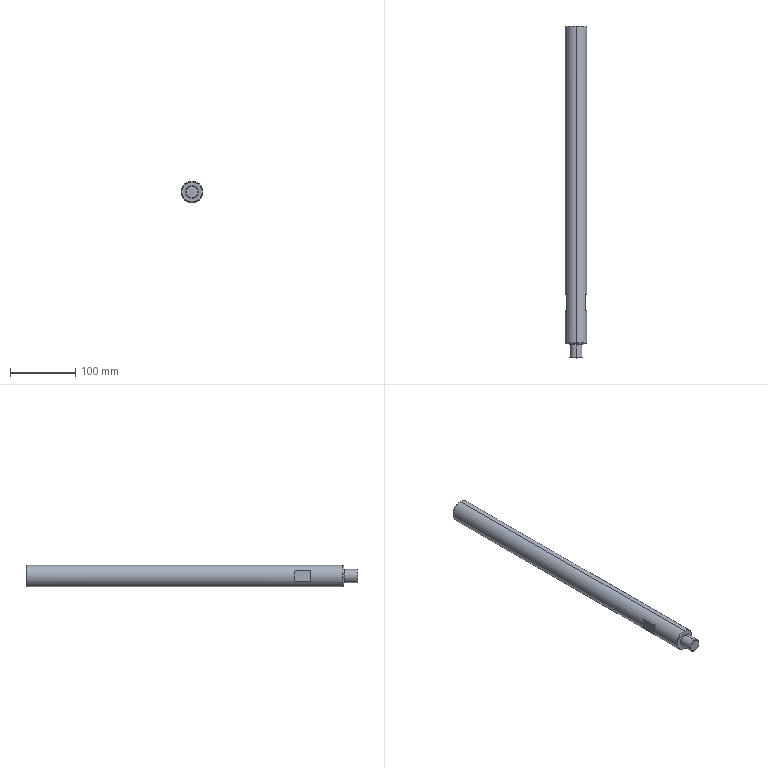Component | SolidWorks | 012A-20130717-1 | 1 solid | 28 faces | box 33 x 508 x 33 mm | volume 408981 mm3 | cone 10 | plane 10 | cylinder 8 | commonest cylinder face diameters 17.5 x2 18 x2 20 x2 33 x2
build123d program:
from build123d import *

# Parameters (mm, degrees)
M20_TAPPED_HOLE1_D     = 17.5
M20_TAPPED_HOLE1_DEPTH = 47.5
M20_TAPPED_HOLE1_TIP   = 5.258
CHAMFER1_SIZE          = 1
CHAMFER2_SIZE          = 1
SKETCH5_OUTSIDE_W      = 137.028
SKETCH5_OUTSIDE_H      = 137.028
SKETCH5_OUTSIDE_W_2    = 41.855
SKETCH5_OUTSIDE_H_2    = 28
CUT_EXTRUDE1_DEPTH     = 25


with BuildPart() as part:
    # Sketch1 → Revolve1 (revolve)
    with BuildSketch(Plane.XY, mode=Mode.PRIVATE) as revolve1_sk:
        Polygon((0, 0), (0, 10), (20, 10), (20, 9), (22, 9), (22, 16.5), (508, 16.5), (508, 0), align=None)
    revolve(revolve1_sk.sketch.rotate(Axis((0, 0, 0), (1, 0, 0)), 90), axis=Axis((0, 0, 0), (1, 0, 0)))

    # M20 Tapped Hole1
    with Locations(Plane(origin=(508, 0, 0), x_dir=(0, 0, 1), z_dir=(1, 0, 0))):
        with Locations((0, 0)):
            Hole(M20_TAPPED_HOLE1_D / 2, depth=M20_TAPPED_HOLE1_DEPTH)
            with Locations((0, 0, -(M20_TAPPED_HOLE1_DEPTH + M20_TAPPED_HOLE1_TIP / 2))):  # 118° drill point
                Cone(0, M20_TAPPED_HOLE1_D / 2, M20_TAPPED_HOLE1_TIP, mode=Mode.SUBTRACT)

    # Chamfer1
    chamfer1_edges = [part.edges().sort_by_distance(p)[0] for p in [
        (0, 0, -10),
    ]]
    chamfer(chamfer1_edges, length=CHAMFER1_SIZE)

    # Chamfer2
    chamfer2_edges = [part.edges().sort_by_distance(p)[0] for p in [
        (508, 0, 8.75),
        (508, 0, -16.5),
        (22, 0, -16.5),
    ]]
    chamfer(chamfer2_edges, length=CHAMFER2_SIZE)

    # Sketch5 outside → Cut-Extrude1 (cut)
    with BuildSketch(Plane.ZY.offset(-72)):
        Rectangle(SKETCH5_OUTSIDE_W, SKETCH5_OUTSIDE_H)
        Rectangle(SKETCH5_OUTSIDE_W_2, SKETCH5_OUTSIDE_H_2, mode=Mode.SUBTRACT)
    extrude(amount=-CUT_EXTRUDE1_DEPTH, mode=Mode.SUBTRACT)


solid = part.part

# Placed as in the assembly
solid = solid.moved(Location((-240, 407.253, 90), (0, 0, 90)))
STEP:
#1=CARTESIAN_POINT('',(-9.449,16.9,4.154));
#2=VERTEX_POINT('',#1);
#3=CARTESIAN_POINT('',(-9.449,16.9,2.933));
#4=VERTEX_POINT('',#3);
#5=CARTESIAN_POINT('',(-9.449,16.9,3.543));
#6=DIRECTION('',(0.,-1.,-0.));
#7=DIRECTION('',(0.,0.,-1.));
#8=AXIS2_PLACEMENT_3D('',#5,#6,#7);
#9=CIRCLE('',#8,0.6102);
#10=EDGE_CURVE('',#2,#4,#9,.T.);
#11=ORIENTED_EDGE('',*,*,#10,.F.);
#12=CARTESIAN_POINT('',(-9.449,16.939,4.193));
#13=VERTEX_POINT('',#12);
#14=CARTESIAN_POINT('',(-9.449,16.9,4.154));
#15=DIRECTION('',(-0.,0.7071,0.7071));
#16=VECTOR('',#15,39.37);
#17=LINE('',#14,#16);
#18=EDGE_CURVE('',#2,#13,#17,.T.);
#19=ORIENTED_EDGE('',*,*,#18,.T.);
#20=CARTESIAN_POINT('',(-9.449,16.939,2.894));
#21=VERTEX_POINT('',#20);
#22=CARTESIAN_POINT('',(-9.449,16.939,3.543));
#23=DIRECTION('',(0.,1.,0.));
#24=DIRECTION('',(0.,0.,-1.));
#25=AXIS2_PLACEMENT_3D('',#22,#23,#24);
#26=CIRCLE('',#25,0.6496);
#27=EDGE_CURVE('',#21,#13,#26,.T.);
#28=ORIENTED_EDGE('',*,*,#27,.F.);
#29=CARTESIAN_POINT('',(-9.449,16.9,2.933));
#30=DIRECTION('',(0.,0.7071,-0.7071));
#31=VECTOR('',#30,39.37);
#32=LINE('',#29,#31);
#33=EDGE_CURVE('',#4,#21,#32,.T.);
#34=ORIENTED_EDGE('',*,*,#33,.F.);
#35=EDGE_LOOP('',(#11,#19,#28,#34));
#36=FACE_OUTER_BOUND('',#35,.T.);
#37=CARTESIAN_POINT('',(-9.449,16.9,3.543));
#38=DIRECTION('',(0.,1.,0.));
#39=DIRECTION('',(0.,0.,-1.));
#40=AXIS2_PLACEMENT_3D('',#37,#38,#39);
#41=CONICAL_SURFACE('',#40,0.6102,0.7854);
#42=ADVANCED_FACE('',(#36),#41,.T.);
#43=CARTESIAN_POINT('',(-9.449,36.034,2.933));
#44=VERTEX_POINT('',#43);
#45=CARTESIAN_POINT('',(-9.449,36.034,4.154));
#46=VERTEX_POINT('',#45);
#47=CARTESIAN_POINT('',(-9.449,36.034,3.543));
#48=DIRECTION('',(0.,1.,0.));
#49=DIRECTION('',(0.,0.,1.));
#50=AXIS2_PLACEMENT_3D('',#47,#48,#49);
#51=CIRCLE('',#50,0.6102);
#52=EDGE_CURVE('',#44,#46,#51,.T.);
#53=ORIENTED_EDGE('',*,*,#52,.F.);
#54=CARTESIAN_POINT('',(-9.449,35.994,2.894));
#55=VERTEX_POINT('',#54);
#56=CARTESIAN_POINT('',(-9.449,35.994,2.894));
#57=DIRECTION('',(-0.,-0.7071,-0.7071));
#58=VECTOR('',#57,39.37);
#59=LINE('',#56,#58);
#60=EDGE_CURVE('',#44,#55,#59,.T.);
#61=ORIENTED_EDGE('',*,*,#60,.T.);
#62=CARTESIAN_POINT('',(-9.449,35.994,4.193));
#63=VERTEX_POINT('',#62);
#64=CARTESIAN_POINT('',(-9.449,35.994,3.543));
#65=DIRECTION('',(0.,-1.,-0.));
#66=DIRECTION('',(0.,0.,1.));
#67=AXIS2_PLACEMENT_3D('',#64,#65,#66);
#68=CIRCLE('',#67,0.6496);
#69=EDGE_CURVE('',#63,#55,#68,.T.);
#70=ORIENTED_EDGE('',*,*,#69,.F.);
#71=CARTESIAN_POINT('',(-9.449,35.994,4.193));
#72=DIRECTION('',(-0.,-0.7071,0.7071));
#73=VECTOR('',#72,39.37);
#74=LINE('',#71,#73);
#75=EDGE_CURVE('',#46,#63,#74,.T.);
#76=ORIENTED_EDGE('',*,*,#75,.F.);
#77=EDGE_LOOP('',(#53,#61,#70,#76));
#78=FACE_OUTER_BOUND('',#77,.T.);
#79=CARTESIAN_POINT('',(-9.449,35.994,3.543));
#80=DIRECTION('',(0.,-1.,-0.));
#81=DIRECTION('',(0.,0.,1.));
#82=AXIS2_PLACEMENT_3D('',#79,#80,#81);
#83=CONICAL_SURFACE('',#82,0.6496,0.7854);
#84=ADVANCED_FACE('',(#78),#83,.T.);
#85=CARTESIAN_POINT('',(-9.449,35.994,3.888));
#86=VERTEX_POINT('',#85);
#87=CARTESIAN_POINT('',(-9.449,35.994,3.199));
#88=VERTEX_POINT('',#87);
#89=CARTESIAN_POINT('',(-9.449,35.994,3.543));
#90=DIRECTION('',(0.,1.,0.));
#91=DIRECTION('',(0.,0.,1.));
#92=AXIS2_PLACEMENT_3D('',#89,#90,#91);
#93=CIRCLE('',#92,0.3445);
#94=EDGE_CURVE('',#86,#88,#93,.T.);
#95=ORIENTED_EDGE('',*,*,#94,.F.);
#96=CARTESIAN_POINT('',(-9.449,36.034,3.927));
#97=VERTEX_POINT('',#96);
#98=CARTESIAN_POINT('',(-9.449,35.994,3.888));
#99=DIRECTION('',(-0.,0.7071,0.7071));
#100=VECTOR('',#99,39.37);
#101=LINE('',#98,#100);
#102=EDGE_CURVE('',#86,#97,#101,.T.);
#103=ORIENTED_EDGE('',*,*,#102,.T.);
#104=CARTESIAN_POINT('',(-9.449,36.034,3.159));
#105=VERTEX_POINT('',#104);
#106=CARTESIAN_POINT('',(-9.449,36.034,3.543));
#107=DIRECTION('',(0.,-1.,-0.));
#108=DIRECTION('',(0.,0.,1.));
#109=AXIS2_PLACEMENT_3D('',#106,#107,#108);
#110=CIRCLE('',#109,0.3839);
#111=EDGE_CURVE('',#105,#97,#110,.T.);
#112=ORIENTED_EDGE('',*,*,#111,.F.);
#113=CARTESIAN_POINT('',(-9.449,35.994,3.199));
#114=DIRECTION('',(0.,0.7071,-0.7071));
#115=VECTOR('',#114,39.37);
#116=LINE('',#113,#115);
#117=EDGE_CURVE('',#88,#105,#116,.T.);
#118=ORIENTED_EDGE('',*,*,#117,.F.);
#119=EDGE_LOOP('',(#95,#103,#112,#118));
#120=FACE_OUTER_BOUND('',#119,.T.);
#121=CARTESIAN_POINT('',(-9.449,35.994,3.543));
#122=DIRECTION('',(0.,1.,0.));
#123=DIRECTION('',(0.,0.,-1.));
#124=AXIS2_PLACEMENT_3D('',#121,#122,#123);
#125=CONICAL_SURFACE('',#124,0.3445,0.7854);
#126=ADVANCED_FACE('',(#120),#125,.F.);
#127=CARTESIAN_POINT('',(-9.449,16.034,3.898));
#128=VERTEX_POINT('',#127);
#129=CARTESIAN_POINT('',(-9.449,16.034,3.189));
#130=VERTEX_POINT('',#129);
#131=CARTESIAN_POINT('',(-9.449,16.034,3.543));
#132=DIRECTION('',(0.,-1.,-0.));
#133=DIRECTION('',(0.,0.,-1.));
#134=AXIS2_PLACEMENT_3D('',#131,#132,#133);
#135=CIRCLE('',#134,0.3543);
#136=EDGE_CURVE('',#128,#130,#135,.T.);
#137=ORIENTED_EDGE('',*,*,#136,.F.);
#138=CARTESIAN_POINT('',(-9.449,16.073,3.937));
#139=VERTEX_POINT('',#138);
#140=CARTESIAN_POINT('',(-9.449,16.034,3.898));
#141=DIRECTION('',(-0.,0.7071,0.7071));
#142=VECTOR('',#141,39.37);
#143=LINE('',#140,#142);
#144=EDGE_CURVE('',#128,#139,#143,.T.);
#145=ORIENTED_EDGE('',*,*,#144,.T.);
#146=CARTESIAN_POINT('',(-9.449,16.073,3.15));
#147=VERTEX_POINT('',#146);
#148=CARTESIAN_POINT('',(-9.449,16.073,3.543));
#149=DIRECTION('',(0.,1.,0.));
#150=DIRECTION('',(0.,0.,-1.));
#151=AXIS2_PLACEMENT_3D('',#148,#149,#150);
#152=CIRCLE('',#151,0.3937);
#153=EDGE_CURVE('',#147,#139,#152,.T.);
#154=ORIENTED_EDGE('',*,*,#153,.F.);
#155=CARTESIAN_POINT('',(-9.449,16.034,3.189));
#156=DIRECTION('',(0.,0.7071,-0.7071));
#157=VECTOR('',#156,39.37);
#158=LINE('',#155,#157);
#159=EDGE_CURVE('',#130,#147,#158,.T.);
#160=ORIENTED_EDGE('',*,*,#159,.F.);
#161=EDGE_LOOP('',(#137,#145,#154,#160));
#162=FACE_OUTER_BOUND('',#161,.T.);
#163=CARTESIAN_POINT('',(-9.449,16.034,3.543));
#164=DIRECTION('',(0.,1.,0.));
#165=DIRECTION('',(0.,0.,-1.));
#166=AXIS2_PLACEMENT_3D('',#163,#164,#165);
#167=CONICAL_SURFACE('',#166,0.3543,0.7854);
#168=ADVANCED_FACE('',(#162),#167,.T.);
#169=CARTESIAN_POINT('',(-9.449,34.164,3.888));
#170=VERTEX_POINT('',#169);
#171=CARTESIAN_POINT('',(-9.449,34.164,3.199));
#172=VERTEX_POINT('',#171);
#173=CARTESIAN_POINT('',(-9.449,34.164,3.543));
#174=DIRECTION('',(0.,1.,0.));
#175=DIRECTION('',(0.,0.,-1.));
#176=AXIS2_PLACEMENT_3D('',#173,#174,#175);
#177=CIRCLE('',#176,0.3445);
#178=EDGE_CURVE('',#170,#172,#177,.T.);
#179=ORIENTED_EDGE('',*,*,#178,.F.);
#180=CARTESIAN_POINT('',(-9.449,36.034,3.888));
#181=DIRECTION('',(0.,1.,0.));
#182=VECTOR('',#181,39.37);
#183=LINE('',#180,#182);
#184=EDGE_CURVE('',#170,#86,#183,.T.);
#185=ORIENTED_EDGE('',*,*,#184,.T.);
#186=ORIENTED_EDGE('',*,*,#94,.T.);
#187=CARTESIAN_POINT('',(-9.449,36.034,3.199));
#188=DIRECTION('',(0.,1.,0.));
#189=VECTOR('',#188,39.37);
#190=LINE('',#187,#189);
#191=EDGE_CURVE('',#172,#88,#190,.T.);
#192=ORIENTED_EDGE('',*,*,#191,.F.);
#193=EDGE_LOOP('',(#179,#185,#186,#192));
#194=FACE_OUTER_BOUND('',#193,.T.);
#195=CARTESIAN_POINT('',(-9.449,36.034,3.543));
#196=DIRECTION('',(0.,1.,0.));
#197=DIRECTION('',(0.,0.,-1.));
#198=AXIS2_PLACEMENT_3D('',#195,#196,#197);
#199=CYLINDRICAL_SURFACE('',#198,0.3445);
#200=ADVANCED_FACE('',(#194),#199,.F.);
#201=CARTESIAN_POINT('',(-9.449,33.957,3.543));
#202=VERTEX_POINT('',#201);
#203=CARTESIAN_POINT('',(-9.449,34.164,3.199));
#204=DIRECTION('',(0.,0.515,-0.8572));
#205=VECTOR('',#204,39.37);
#206=LINE('',#203,#205);
#207=EDGE_CURVE('',#202,#172,#206,.T.);
#208=ORIENTED_EDGE('',*,*,#207,.F.);
#209=CARTESIAN_POINT('',(-9.449,34.164,3.888));
#210=DIRECTION('',(-0.,0.515,0.8572));
#211=VECTOR('',#210,39.37);
#212=LINE('',#209,#211);
#213=EDGE_CURVE('',#202,#170,#212,.T.);
#214=ORIENTED_EDGE('',*,*,#213,.T.);
#215=ORIENTED_EDGE('',*,*,#178,.T.);
#216=EDGE_LOOP('',(#208,#214,#215));
#217=FACE_OUTER_BOUND('',#216,.T.);
#218=CARTESIAN_POINT('',(-9.449,34.164,3.543));
#219=DIRECTION('',(0.,1.,0.));
#220=DIRECTION('',(0.,0.,-1.));
#221=AXIS2_PLACEMENT_3D('',#218,#219,#220);
#222=CONICAL_SURFACE('',#221,0.3445,1.03);
#223=ADVANCED_FACE('',(#217),#222,.F.);
#224=CARTESIAN_POINT('',(-9.449,16.9,3.898));
#225=VERTEX_POINT('',#224);
#226=CARTESIAN_POINT('',(-9.449,16.9,3.189));
#227=VERTEX_POINT('',#226);
#228=CARTESIAN_POINT('',(-9.449,16.9,3.543));
#229=DIRECTION('',(0.,-1.,-0.));
#230=DIRECTION('',(0.,0.,1.));
#231=AXIS2_PLACEMENT_3D('',#228,#229,#230);
#232=CIRCLE('',#231,0.3543);
#233=EDGE_CURVE('',#225,#227,#232,.T.);
#234=ORIENTED_EDGE('',*,*,#233,.T.);
#235=CARTESIAN_POINT('',(-9.449,16.821,3.189));
#236=VERTEX_POINT('',#235);
#237=CARTESIAN_POINT('',(-9.449,16.034,3.189));
#238=DIRECTION('',(0.,-1.,-0.));
#239=VECTOR('',#238,39.37);
#240=LINE('',#237,#239);
#241=EDGE_CURVE('',#227,#236,#240,.T.);
#242=ORIENTED_EDGE('',*,*,#241,.T.);
#243=CARTESIAN_POINT('',(-9.449,16.821,3.898));
#244=VERTEX_POINT('',#243);
#245=CARTESIAN_POINT('',(-9.449,16.821,3.543));
#246=DIRECTION('',(0.,-1.,-0.));
#247=DIRECTION('',(0.,0.,1.));
#248=AXIS2_PLACEMENT_3D('',#245,#246,#247);
#249=CIRCLE('',#248,0.3543);
#250=EDGE_CURVE('',#244,#236,#249,.T.);
#251=ORIENTED_EDGE('',*,*,#250,.F.);
#252=CARTESIAN_POINT('',(-9.449,16.034,3.898));
#253=DIRECTION('',(0.,-1.,-0.));
#254=VECTOR('',#253,39.37);
#255=LINE('',#252,#254);
#256=EDGE_CURVE('',#225,#244,#255,.T.);
#257=ORIENTED_EDGE('',*,*,#256,.F.);
#258=EDGE_LOOP('',(#234,#242,#251,#257));
#259=FACE_OUTER_BOUND('',#258,.T.);
#260=CARTESIAN_POINT('',(-9.449,16.034,3.543));
#261=DIRECTION('',(0.,-1.,-0.));
#262=DIRECTION('',(0.,0.,1.));
#263=AXIS2_PLACEMENT_3D('',#260,#261,#262);
#264=CYLINDRICAL_SURFACE('',#263,0.3543);
#265=ADVANCED_FACE('',(#259),#264,.T.);
#266=CARTESIAN_POINT('',(-9.449,16.821,3.937));
#267=VERTEX_POINT('',#266);
#268=CARTESIAN_POINT('',(-9.449,16.821,3.15));
#269=VERTEX_POINT('',#268);
#270=CARTESIAN_POINT('',(-9.449,16.821,3.543));
#271=DIRECTION('',(0.,-1.,-0.));
#272=DIRECTION('',(0.,0.,1.));
#273=AXIS2_PLACEMENT_3D('',#270,#271,#272);
#274=CIRCLE('',#273,0.3937);
#275=EDGE_CURVE('',#267,#269,#274,.T.);
#276=ORIENTED_EDGE('',*,*,#275,.T.);
#277=CARTESIAN_POINT('',(-9.449,16.034,3.15));
#278=DIRECTION('',(0.,-1.,-0.));
#279=VECTOR('',#278,39.37);
#280=LINE('',#277,#279);
#281=EDGE_CURVE('',#269,#147,#280,.T.);
#282=ORIENTED_EDGE('',*,*,#281,.T.);
#283=ORIENTED_EDGE('',*,*,#153,.T.);
#284=CARTESIAN_POINT('',(-9.449,16.034,3.937));
#285=DIRECTION('',(0.,-1.,-0.));
#286=VECTOR('',#285,39.37);
#287=LINE('',#284,#286);
#288=EDGE_CURVE('',#267,#139,#287,.T.);
#289=ORIENTED_EDGE('',*,*,#288,.F.);
#290=EDGE_LOOP('',(#276,#282,#283,#289));
#291=FACE_OUTER_BOUND('',#290,.T.);
#292=CARTESIAN_POINT('',(-9.449,16.034,3.543));
#293=DIRECTION('',(0.,-1.,-0.));
#294=DIRECTION('',(0.,0.,1.));
#295=AXIS2_PLACEMENT_3D('',#292,#293,#294);
#296=CYLINDRICAL_SURFACE('',#295,0.3937);
#297=ADVANCED_FACE('',(#291),#296,.T.);
#298=CARTESIAN_POINT('',(-10.,19.852,3.2));
#299=VERTEX_POINT('',#298);
#300=CARTESIAN_POINT('',(-10.,18.868,3.2));
#301=VERTEX_POINT('',#300);
#302=CARTESIAN_POINT('',(-10.,16.034,3.2));
#303=DIRECTION('',(0.,-1.,-0.));
#304=VECTOR('',#303,39.37);
#305=LINE('',#302,#304);
#306=EDGE_CURVE('',#299,#301,#305,.T.);
#307=ORIENTED_EDGE('',*,*,#306,.F.);
#308=CARTESIAN_POINT('',(-10.,19.852,3.887));
#309=VERTEX_POINT('',#308);
#310=CARTESIAN_POINT('',(-9.449,19.852,3.543));
#311=DIRECTION('',(0.,-1.,-0.));
#312=DIRECTION('',(0.,0.,1.));
#313=AXIS2_PLACEMENT_3D('',#310,#311,#312);
#314=CIRCLE('',#313,0.6496);
#315=EDGE_CURVE('',#309,#299,#314,.T.);
#316=ORIENTED_EDGE('',*,*,#315,.F.);
#317=CARTESIAN_POINT('',(-10.,18.868,3.887));
#318=VERTEX_POINT('',#317);
#319=CARTESIAN_POINT('',(-10.,16.034,3.887));
#320=DIRECTION('',(0.,1.,0.));
#321=VECTOR('',#320,39.37);
#322=LINE('',#319,#321);
#323=EDGE_CURVE('',#318,#309,#322,.T.);
#324=ORIENTED_EDGE('',*,*,#323,.F.);
#325=CARTESIAN_POINT('',(-9.449,18.868,3.543));
#326=DIRECTION('',(0.,-1.,-0.));
#327=DIRECTION('',(0.,0.,1.));
#328=AXIS2_PLACEMENT_3D('',#325,#326,#327);
#329=CIRCLE('',#328,0.6496);
#330=EDGE_CURVE('',#318,#301,#329,.T.);
#331=ORIENTED_EDGE('',*,*,#330,.T.);
#332=EDGE_LOOP('',(#307,#316,#324,#331));
#333=FACE_BOUND('',#332,.T.);
#334=ORIENTED_EDGE('',*,*,#69,.T.);
#335=CARTESIAN_POINT('',(-9.449,16.034,2.894));
#336=DIRECTION('',(0.,-1.,-0.));
#337=VECTOR('',#336,39.37);
#338=LINE('',#335,#337);
#339=EDGE_CURVE('',#55,#21,#338,.T.);
#340=ORIENTED_EDGE('',*,*,#339,.T.);
#341=ORIENTED_EDGE('',*,*,#27,.T.);
#342=CARTESIAN_POINT('',(-9.449,16.034,4.193));
#343=DIRECTION('',(0.,-1.,-0.));
#344=VECTOR('',#343,39.37);
#345=LINE('',#342,#344);
#346=EDGE_CURVE('',#63,#13,#345,.T.);
#347=ORIENTED_EDGE('',*,*,#346,.F.);
#348=EDGE_LOOP('',(#334,#340,#341,#347));
#349=FACE_OUTER_BOUND('',#348,.T.);
#350=CARTESIAN_POINT('',(-9.449,16.034,3.543));
#351=DIRECTION('',(0.,-1.,-0.));
#352=DIRECTION('',(0.,0.,1.));
#353=AXIS2_PLACEMENT_3D('',#350,#351,#352);
#354=CYLINDRICAL_SURFACE('',#353,0.6496);
#355=ADVANCED_FACE('',(#333,#349),#354,.T.);
#356=ORIENTED_EDGE('',*,*,#339,.F.);
#357=CARTESIAN_POINT('',(-9.449,35.994,3.543));
#358=DIRECTION('',(0.,-1.,-0.));
#359=DIRECTION('',(0.,0.,1.));
#360=AXIS2_PLACEMENT_3D('',#357,#358,#359);
#361=CIRCLE('',#360,0.6496);
#362=EDGE_CURVE('',#55,#63,#361,.T.);
#363=ORIENTED_EDGE('',*,*,#362,.T.);
#364=ORIENTED_EDGE('',*,*,#346,.T.);
#365=CARTESIAN_POINT('',(-9.449,16.939,3.543));
#366=DIRECTION('',(0.,1.,0.));
#367=DIRECTION('',(0.,0.,-1.));
#368=AXIS2_PLACEMENT_3D('',#365,#366,#367);
#369=CIRCLE('',#368,0.6496);
#370=EDGE_CURVE('',#13,#21,#369,.T.);
#371=ORIENTED_EDGE('',*,*,#370,.T.);
#372=EDGE_LOOP('',(#356,#363,#364,#371));
#373=FACE_OUTER_BOUND('',#372,.T.);
#374=CARTESIAN_POINT('',(-8.898,19.852,3.887));
#375=VERTEX_POINT('',#374);
#376=CARTESIAN_POINT('',(-8.898,18.868,3.887));
#377=VERTEX_POINT('',#376);
#378=CARTESIAN_POINT('',(-8.898,16.034,3.887));
#379=DIRECTION('',(0.,-1.,-0.));
#380=VECTOR('',#379,39.37);
#381=LINE('',#378,#380);
#382=EDGE_CURVE('',#375,#377,#381,.T.);
#383=ORIENTED_EDGE('',*,*,#382,.F.);
#384=CARTESIAN_POINT('',(-8.898,19.852,3.2));
#385=VERTEX_POINT('',#384);
#386=CARTESIAN_POINT('',(-9.449,19.852,3.543));
#387=DIRECTION('',(0.,-1.,-0.));
#388=DIRECTION('',(0.,0.,1.));
#389=AXIS2_PLACEMENT_3D('',#386,#387,#388);
#390=CIRCLE('',#389,0.6496);
#391=EDGE_CURVE('',#385,#375,#390,.T.);
#392=ORIENTED_EDGE('',*,*,#391,.F.);
#393=CARTESIAN_POINT('',(-8.898,18.868,3.2));
#394=VERTEX_POINT('',#393);
#395=CARTESIAN_POINT('',(-8.898,16.034,3.2));
#396=DIRECTION('',(0.,1.,0.));
#397=VECTOR('',#396,39.37);
#398=LINE('',#395,#397);
#399=EDGE_CURVE('',#394,#385,#398,.T.);
#400=ORIENTED_EDGE('',*,*,#399,.F.);
#401=CARTESIAN_POINT('',(-9.449,18.868,3.543));
#402=DIRECTION('',(0.,-1.,-0.));
#403=DIRECTION('',(0.,0.,1.));
#404=AXIS2_PLACEMENT_3D('',#401,#402,#403);
#405=CIRCLE('',#404,0.6496);
#406=EDGE_CURVE('',#394,#377,#405,.T.);
#407=ORIENTED_EDGE('',*,*,#406,.T.);
#408=EDGE_LOOP('',(#383,#392,#400,#407));
#409=FACE_BOUND('',#408,.T.);
#410=CARTESIAN_POINT('',(-9.449,16.034,3.543));
#411=DIRECTION('',(0.,-1.,-0.));
#412=DIRECTION('',(0.,0.,1.));
#413=AXIS2_PLACEMENT_3D('',#410,#411,#412);
#414=CYLINDRICAL_SURFACE('',#413,0.6496);
#415=ADVANCED_FACE('',(#373,#409),#414,.T.);
#416=CARTESIAN_POINT('',(-9.449,16.034,3.543));
#417=DIRECTION('',(0.,-1.,-0.));
#418=DIRECTION('',(0.,0.,-1.));
#419=AXIS2_PLACEMENT_3D('',#416,#417,#418);
#420=CIRCLE('',#419,0.3543);
#421=EDGE_CURVE('',#130,#128,#420,.T.);
#422=ORIENTED_EDGE('',*,*,#421,.T.);
#423=ORIENTED_EDGE('',*,*,#136,.T.);
#424=EDGE_LOOP('',(#422,#423));
#425=FACE_OUTER_BOUND('',#424,.T.);
#426=CARTESIAN_POINT('',(-9.449,16.034,3.543));
#427=DIRECTION('',(0.,1.,0.));
#428=DIRECTION('',(0.,0.,-1.));
#429=AXIS2_PLACEMENT_3D('',#426,#427,#428);
#430=PLANE('',#429);
#431=ADVANCED_FACE('',(#425),#430,.F.);
#432=ORIENTED_EDGE('',*,*,#281,.F.);
#433=CARTESIAN_POINT('',(-9.449,16.821,3.543));
#434=DIRECTION('',(0.,-1.,-0.));
#435=DIRECTION('',(0.,0.,1.));
#436=AXIS2_PLACEMENT_3D('',#433,#434,#435);
#437=CIRCLE('',#436,0.3937);
#438=EDGE_CURVE('',#269,#267,#437,.T.);
#439=ORIENTED_EDGE('',*,*,#438,.T.);
#440=ORIENTED_EDGE('',*,*,#288,.T.);
#441=CARTESIAN_POINT('',(-9.449,16.073,3.543));
#442=DIRECTION('',(0.,1.,0.));
#443=DIRECTION('',(0.,0.,-1.));
#444=AXIS2_PLACEMENT_3D('',#441,#442,#443);
#445=CIRCLE('',#444,0.3937);
#446=EDGE_CURVE('',#139,#147,#445,.T.);
#447=ORIENTED_EDGE('',*,*,#446,.T.);
#448=EDGE_LOOP('',(#432,#439,#440,#447));
#449=FACE_OUTER_BOUND('',#448,.T.);
#450=CARTESIAN_POINT('',(-9.449,16.034,3.543));
#451=DIRECTION('',(0.,-1.,-0.));
#452=DIRECTION('',(0.,0.,1.));
#453=AXIS2_PLACEMENT_3D('',#450,#451,#452);
#454=CYLINDRICAL_SURFACE('',#453,0.3937);
#455=ADVANCED_FACE('',(#449),#454,.T.);
#456=ORIENTED_EDGE('',*,*,#275,.F.);
#457=ORIENTED_EDGE('',*,*,#438,.F.);
#458=EDGE_LOOP('',(#456,#457));
#459=FACE_OUTER_BOUND('',#458,.T.);
#460=ORIENTED_EDGE('',*,*,#250,.T.);
#461=CARTESIAN_POINT('',(-9.449,16.821,3.543));
#462=DIRECTION('',(0.,-1.,-0.));
#463=DIRECTION('',(0.,0.,1.));
#464=AXIS2_PLACEMENT_3D('',#461,#462,#463);
#465=CIRCLE('',#464,0.3543);
#466=EDGE_CURVE('',#236,#244,#465,.T.);
#467=ORIENTED_EDGE('',*,*,#466,.T.);
#468=EDGE_LOOP('',(#460,#467));
#469=FACE_BOUND('',#468,.T.);
#470=CARTESIAN_POINT('',(-9.843,16.821,3.543));
#471=DIRECTION('',(0.,-1.,-0.));
#472=DIRECTION('',(-0.,-0.,1.));
#473=AXIS2_PLACEMENT_3D('',#470,#471,#472);
#474=PLANE('',#473);
#475=ADVANCED_FACE('',(#459,#469),#474,.F.);
#476=ORIENTED_EDGE('',*,*,#241,.F.);
#477=CARTESIAN_POINT('',(-9.449,16.9,3.543));
#478=DIRECTION('',(0.,-1.,-0.));
#479=DIRECTION('',(0.,0.,1.));
#480=AXIS2_PLACEMENT_3D('',#477,#478,#479);
#481=CIRCLE('',#480,0.3543);
#482=EDGE_CURVE('',#227,#225,#481,.T.);
#483=ORIENTED_EDGE('',*,*,#482,.T.);
#484=ORIENTED_EDGE('',*,*,#256,.T.);
#485=ORIENTED_EDGE('',*,*,#466,.F.);
#486=EDGE_LOOP('',(#476,#483,#484,#485));
#487=FACE_OUTER_BOUND('',#486,.T.);
#488=CARTESIAN_POINT('',(-9.449,16.034,3.543));
#489=DIRECTION('',(0.,-1.,-0.));
#490=DIRECTION('',(0.,0.,1.));
#491=AXIS2_PLACEMENT_3D('',#488,#489,#490);
#492=CYLINDRICAL_SURFACE('',#491,0.3543);
#493=ADVANCED_FACE('',(#487),#492,.T.);
#494=CARTESIAN_POINT('',(-9.449,16.9,3.543));
#495=DIRECTION('',(0.,-1.,-0.));
#496=DIRECTION('',(0.,0.,-1.));
#497=AXIS2_PLACEMENT_3D('',#494,#495,#496);
#498=CIRCLE('',#497,0.6102);
#499=EDGE_CURVE('',#4,#2,#498,.T.);
#500=ORIENTED_EDGE('',*,*,#499,.T.);
#501=ORIENTED_EDGE('',*,*,#10,.T.);
#502=EDGE_LOOP('',(#500,#501));
#503=FACE_OUTER_BOUND('',#502,.T.);
#504=ORIENTED_EDGE('',*,*,#233,.F.);
#505=ORIENTED_EDGE('',*,*,#482,.F.);
#506=EDGE_LOOP('',(#504,#505));
#507=FACE_BOUND('',#506,.T.);
#508=CARTESIAN_POINT('',(-9.803,16.9,3.543));
#509=DIRECTION('',(0.,1.,0.));
#510=DIRECTION('',(0.,0.,-1.));
#511=AXIS2_PLACEMENT_3D('',#508,#509,#510);
#512=PLANE('',#511);
#513=ADVANCED_FACE('',(#503,#507),#512,.F.);
#514=ORIENTED_EDGE('',*,*,#111,.T.);
#515=CARTESIAN_POINT('',(-9.449,36.034,3.543));
#516=DIRECTION('',(0.,-1.,-0.));
#517=DIRECTION('',(0.,0.,1.));
#518=AXIS2_PLACEMENT_3D('',#515,#516,#517);
#519=CIRCLE('',#518,0.3839);
#520=EDGE_CURVE('',#97,#105,#519,.T.);
#521=ORIENTED_EDGE('',*,*,#520,.T.);
#522=EDGE_LOOP('',(#514,#521));
#523=FACE_BOUND('',#522,.T.);
#524=CARTESIAN_POINT('',(-9.449,36.034,3.543));
#525=DIRECTION('',(0.,1.,0.));
#526=DIRECTION('',(0.,0.,1.));
#527=AXIS2_PLACEMENT_3D('',#524,#525,#526);
#528=CIRCLE('',#527,0.6102);
#529=EDGE_CURVE('',#46,#44,#528,.T.);
#530=ORIENTED_EDGE('',*,*,#529,.T.);
#531=ORIENTED_EDGE('',*,*,#52,.T.);
#532=EDGE_LOOP('',(#530,#531));
#533=FACE_OUTER_BOUND('',#532,.T.);
#534=CARTESIAN_POINT('',(-10.098,36.034,3.543));
#535=DIRECTION('',(0.,-1.,-0.));
#536=DIRECTION('',(-0.,-0.,1.));
#537=AXIS2_PLACEMENT_3D('',#534,#535,#536);
#538=PLANE('',#537);
#539=ADVANCED_FACE('',(#523,#533),#538,.F.);
#540=ORIENTED_EDGE('',*,*,#213,.F.);
#541=ORIENTED_EDGE('',*,*,#207,.T.);
#542=CARTESIAN_POINT('',(-9.449,34.164,3.543));
#543=DIRECTION('',(0.,1.,0.));
#544=DIRECTION('',(0.,0.,-1.));
#545=AXIS2_PLACEMENT_3D('',#542,#543,#544);
#546=CIRCLE('',#545,0.3445);
#547=EDGE_CURVE('',#172,#170,#546,.T.);
#548=ORIENTED_EDGE('',*,*,#547,.T.);
#549=EDGE_LOOP('',(#540,#541,#548));
#550=FACE_OUTER_BOUND('',#549,.T.);
#551=CARTESIAN_POINT('',(-9.449,34.164,3.543));
#552=DIRECTION('',(0.,1.,0.));
#553=DIRECTION('',(0.,0.,-1.));
#554=AXIS2_PLACEMENT_3D('',#551,#552,#553);
#555=CONICAL_SURFACE('',#554,0.3445,1.03);
#556=ADVANCED_FACE('',(#550),#555,.F.);
#557=ORIENTED_EDGE('',*,*,#184,.F.);
#558=ORIENTED_EDGE('',*,*,#547,.F.);
#559=ORIENTED_EDGE('',*,*,#191,.T.);
#560=CARTESIAN_POINT('',(-9.449,35.994,3.543));
#561=DIRECTION('',(0.,1.,0.));
#562=DIRECTION('',(0.,0.,1.));
#563=AXIS2_PLACEMENT_3D('',#560,#561,#562);
#564=CIRCLE('',#563,0.3445);
#565=EDGE_CURVE('',#88,#86,#564,.T.);
#566=ORIENTED_EDGE('',*,*,#565,.T.);
#567=EDGE_LOOP('',(#557,#558,#559,#566));
#568=FACE_OUTER_BOUND('',#567,.T.);
#569=CARTESIAN_POINT('',(-9.449,36.034,3.543));
#570=DIRECTION('',(0.,1.,0.));
#571=DIRECTION('',(0.,0.,-1.));
#572=AXIS2_PLACEMENT_3D('',#569,#570,#571);
#573=CYLINDRICAL_SURFACE('',#572,0.3445);
#574=ADVANCED_FACE('',(#568),#573,.F.);
#575=ORIENTED_EDGE('',*,*,#144,.F.);
#576=ORIENTED_EDGE('',*,*,#421,.F.);
#577=ORIENTED_EDGE('',*,*,#159,.T.);
#578=ORIENTED_EDGE('',*,*,#446,.F.);
#579=EDGE_LOOP('',(#575,#576,#577,#578));
#580=FACE_OUTER_BOUND('',#579,.T.);
#581=CARTESIAN_POINT('',(-9.449,16.034,3.543));
#582=DIRECTION('',(0.,1.,0.));
#583=DIRECTION('',(0.,0.,-1.));
#584=AXIS2_PLACEMENT_3D('',#581,#582,#583);
#585=CONICAL_SURFACE('',#584,0.3543,0.7854);
#586=ADVANCED_FACE('',(#580),#585,.T.);
#587=ORIENTED_EDGE('',*,*,#102,.F.);
#588=ORIENTED_EDGE('',*,*,#565,.F.);
#589=ORIENTED_EDGE('',*,*,#117,.T.);
#590=ORIENTED_EDGE('',*,*,#520,.F.);
#591=EDGE_LOOP('',(#587,#588,#589,#590));
#592=FACE_OUTER_BOUND('',#591,.T.);
#593=CARTESIAN_POINT('',(-9.449,35.994,3.543));
#594=DIRECTION('',(0.,1.,0.));
#595=DIRECTION('',(0.,0.,-1.));
#596=AXIS2_PLACEMENT_3D('',#593,#594,#595);
#597=CONICAL_SURFACE('',#596,0.3445,0.7854);
#598=ADVANCED_FACE('',(#592),#597,.F.);
#599=ORIENTED_EDGE('',*,*,#60,.F.);
#600=ORIENTED_EDGE('',*,*,#529,.F.);
#601=ORIENTED_EDGE('',*,*,#75,.T.);
#602=ORIENTED_EDGE('',*,*,#362,.F.);
#603=EDGE_LOOP('',(#599,#600,#601,#602));
#604=FACE_OUTER_BOUND('',#603,.T.);
#605=CARTESIAN_POINT('',(-9.449,35.994,3.543));
#606=DIRECTION('',(0.,-1.,-0.));
#607=DIRECTION('',(0.,0.,1.));
#608=AXIS2_PLACEMENT_3D('',#605,#606,#607);
#609=CONICAL_SURFACE('',#608,0.6496,0.7854);
#610=ADVANCED_FACE('',(#604),#609,.T.);
#611=ORIENTED_EDGE('',*,*,#18,.F.);
#612=ORIENTED_EDGE('',*,*,#499,.F.);
#613=ORIENTED_EDGE('',*,*,#33,.T.);
#614=ORIENTED_EDGE('',*,*,#370,.F.);
#615=EDGE_LOOP('',(#611,#612,#613,#614));
#616=FACE_OUTER_BOUND('',#615,.T.);
#617=CARTESIAN_POINT('',(-9.449,16.9,3.543));
#618=DIRECTION('',(0.,1.,0.));
#619=DIRECTION('',(0.,0.,-1.));
#620=AXIS2_PLACEMENT_3D('',#617,#618,#619);
#621=CONICAL_SURFACE('',#620,0.6102,0.7854);
#622=ADVANCED_FACE('',(#616),#621,.T.);
#623=ORIENTED_EDGE('',*,*,#306,.T.);
#624=CARTESIAN_POINT('',(-10.,18.868,2.719));
#625=DIRECTION('',(0.,0.,-1.));
#626=VECTOR('',#625,39.37);
#627=LINE('',#624,#626);
#628=EDGE_CURVE('',#318,#301,#627,.T.);
#629=ORIENTED_EDGE('',*,*,#628,.F.);
#630=ORIENTED_EDGE('',*,*,#323,.T.);
#631=CARTESIAN_POINT('',(-10.,19.852,2.719));
#632=DIRECTION('',(0.,0.,-1.));
#633=VECTOR('',#632,39.37);
#634=LINE('',#631,#633);
#635=EDGE_CURVE('',#309,#299,#634,.T.);
#636=ORIENTED_EDGE('',*,*,#635,.T.);
#637=EDGE_LOOP('',(#623,#629,#630,#636));
#638=FACE_OUTER_BOUND('',#637,.T.);
#639=CARTESIAN_POINT('',(-10.,19.852,2.719));
#640=DIRECTION('',(-1.,0.,-0.));
#641=DIRECTION('',(-0.,-0.,1.));
#642=AXIS2_PLACEMENT_3D('',#639,#640,#641);
#643=PLANE('',#642);
#644=ADVANCED_FACE('',(#638),#643,.T.);
#645=ORIENTED_EDGE('',*,*,#628,.T.);
#646=ORIENTED_EDGE('',*,*,#330,.F.);
#647=EDGE_LOOP('',(#645,#646));
#648=FACE_OUTER_BOUND('',#647,.T.);
#649=CARTESIAN_POINT('',(-9.449,18.868,3.543));
#650=DIRECTION('',(0.,-1.,-0.));
#651=DIRECTION('',(-0.,-0.,1.));
#652=AXIS2_PLACEMENT_3D('',#649,#650,#651);
#653=PLANE('',#652);
#654=ADVANCED_FACE('',(#648),#653,.F.);
#655=ORIENTED_EDGE('',*,*,#315,.T.);
#656=ORIENTED_EDGE('',*,*,#635,.F.);
#657=EDGE_LOOP('',(#655,#656));
#658=FACE_OUTER_BOUND('',#657,.T.);
#659=CARTESIAN_POINT('',(-9.449,19.852,3.543));
#660=DIRECTION('',(0.,-1.,-0.));
#661=DIRECTION('',(-0.,-0.,1.));
#662=AXIS2_PLACEMENT_3D('',#659,#660,#661);
#663=PLANE('',#662);
#664=ADVANCED_FACE('',(#658),#663,.T.);
#665=ORIENTED_EDGE('',*,*,#391,.T.);
#666=CARTESIAN_POINT('',(-8.898,19.852,2.719));
#667=DIRECTION('',(-0.,-0.,1.));
#668=VECTOR('',#667,39.37);
#669=LINE('',#666,#668);
#670=EDGE_CURVE('',#385,#375,#669,.T.);
#671=ORIENTED_EDGE('',*,*,#670,.F.);
#672=EDGE_LOOP('',(#665,#671));
#673=FACE_OUTER_BOUND('',#672,.T.);
#674=CARTESIAN_POINT('',(-9.449,19.852,3.543));
#675=DIRECTION('',(0.,-1.,-0.));
#676=DIRECTION('',(-0.,-0.,1.));
#677=AXIS2_PLACEMENT_3D('',#674,#675,#676);
#678=PLANE('',#677);
#679=ADVANCED_FACE('',(#673),#678,.T.);
#680=CARTESIAN_POINT('',(-8.898,18.868,2.719));
#681=DIRECTION('',(-0.,-0.,1.));
#682=VECTOR('',#681,39.37);
#683=LINE('',#680,#682);
#684=EDGE_CURVE('',#394,#377,#683,.T.);
#685=ORIENTED_EDGE('',*,*,#684,.T.);
#686=ORIENTED_EDGE('',*,*,#406,.F.);
#687=EDGE_LOOP('',(#685,#686));
#688=FACE_OUTER_BOUND('',#687,.T.);
#689=CARTESIAN_POINT('',(-9.449,18.868,3.543));
#690=DIRECTION('',(0.,-1.,-0.));
#691=DIRECTION('',(-0.,-0.,1.));
#692=AXIS2_PLACEMENT_3D('',#689,#690,#691);
#693=PLANE('',#692);
#694=ADVANCED_FACE('',(#688),#693,.F.);
#695=ORIENTED_EDGE('',*,*,#382,.T.);
#696=ORIENTED_EDGE('',*,*,#684,.F.);
#697=ORIENTED_EDGE('',*,*,#399,.T.);
#698=ORIENTED_EDGE('',*,*,#670,.T.);
#699=EDGE_LOOP('',(#695,#696,#697,#698));
#700=FACE_OUTER_BOUND('',#699,.T.);
#701=CARTESIAN_POINT('',(-8.898,19.852,2.719));
#702=DIRECTION('',(1.,-0.,0.));
#703=DIRECTION('',(0.,0.,-1.));
#704=AXIS2_PLACEMENT_3D('',#701,#702,#703);
#705=PLANE('',#704);
#706=ADVANCED_FACE('',(#700),#705,.T.);
#707=CLOSED_SHELL('',(#42,#84,#126,#168,#200,#223,#265,#297,#355,#415,#431,#455,#475,#493,#513,#539,#556,#574,#586,#598,#610,#622,#644,#654,#664,#679,#694,#706));
#708=MANIFOLD_SOLID_BREP('',#707);
#709=CARTESIAN_POINT('',(0.,0.,0.));
#710=DIRECTION('',(0.,0.,1.));
#711=DIRECTION('',(1.,0.,0.));
#712=AXIS2_PLACEMENT_3D('',#709,#710,#711);
#713=(LENGTH_UNIT()NAMED_UNIT(*)SI_UNIT($,.METRE.));
#714=LENGTH_MEASURE_WITH_UNIT(LENGTH_MEASURE(0.0254),#713);
#715=DIMENSIONAL_EXPONENTS(1.,0.,0.,0.,0.,0.,0.);
#716=(CONVERSION_BASED_UNIT('',#714)LENGTH_UNIT()NAMED_UNIT(#715));
#717=UNCERTAINTY_MEASURE_WITH_UNIT(LENGTH_MEASURE(0.00001),#716,'','');
#718=(NAMED_UNIT(*)PLANE_ANGLE_UNIT()SI_UNIT($,.RADIAN.));
#719=(NAMED_UNIT(*)SI_UNIT($,.STERADIAN.)SOLID_ANGLE_UNIT());
#720=(GEOMETRIC_REPRESENTATION_CONTEXT(3)GLOBAL_UNCERTAINTY_ASSIGNED_CONTEXT((#717))GLOBAL_UNIT_ASSIGNED_CONTEXT((#716,#718,#719))REPRESENTATION_CONTEXT('',''));
#721=ADVANCED_BREP_SHAPE_REPRESENTATION('',(#708,#712),#720);
#722=COLOUR_RGB('',0.7922,0.8196,0.9333);
#723=FILL_AREA_STYLE_COLOUR('',#722);
#724=FILL_AREA_STYLE('',(#723));
#725=SURFACE_STYLE_FILL_AREA(#724);
#726=SURFACE_SIDE_STYLE('',(#725));
#727=SURFACE_STYLE_USAGE(.BOTH.,#726);
#728=PRESENTATION_STYLE_ASSIGNMENT((#727));
#729=STYLED_ITEM('',(#728),#708);
#730=(LENGTH_UNIT()NAMED_UNIT(*)SI_UNIT($,.METRE.));
#731=LENGTH_MEASURE_WITH_UNIT(LENGTH_MEASURE(0.0254),#730);
#732=DIMENSIONAL_EXPONENTS(1.,0.,0.,0.,0.,0.,0.);
#733=(CONVERSION_BASED_UNIT('',#731)LENGTH_UNIT()NAMED_UNIT(#732));
#734=UNCERTAINTY_MEASURE_WITH_UNIT(LENGTH_MEASURE(0.00001),#733,'','');
#735=(NAMED_UNIT(*)PLANE_ANGLE_UNIT()SI_UNIT($,.RADIAN.));
#736=(NAMED_UNIT(*)SI_UNIT($,.STERADIAN.)SOLID_ANGLE_UNIT());
#737=(GEOMETRIC_REPRESENTATION_CONTEXT(3)GLOBAL_UNCERTAINTY_ASSIGNED_CONTEXT((#734))GLOBAL_UNIT_ASSIGNED_CONTEXT((#733,#735,#736))REPRESENTATION_CONTEXT('',''));
#738=MECHANICAL_DESIGN_GEOMETRIC_PRESENTATION_REPRESENTATION('',(#729),#737);
#739=PRESENTATION_LAYER_ASSIGNMENT('','',(#729));